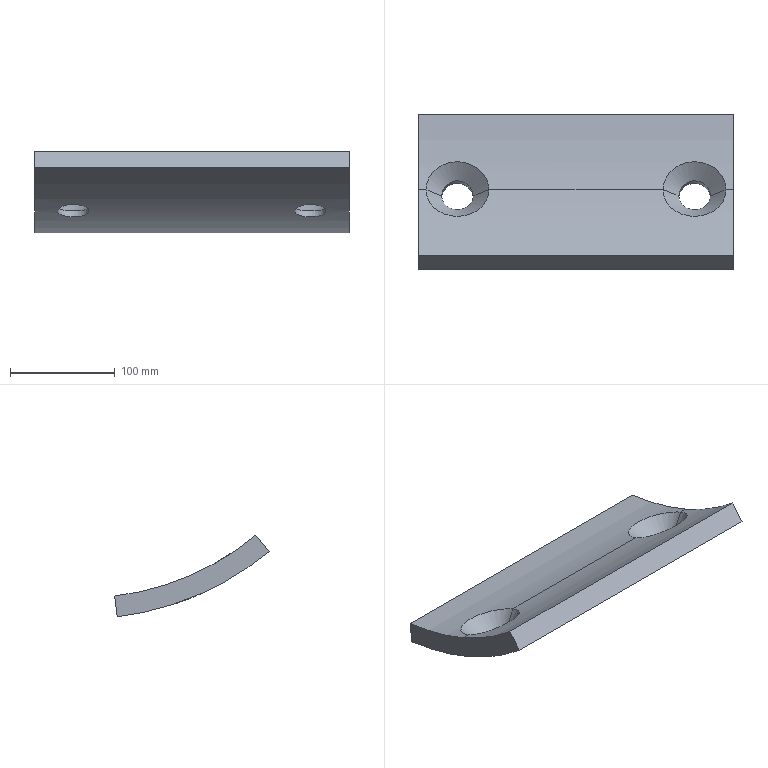Component | SolidWorks | Donja oslona ploca-10_Donja kontaktna ploca-1 | 1 solid | 16 faces | volume 872472 mm3 | cylinder 8 | spline 4 | plane 4 | commonest cylinder face diameters 30 x4 521 x2 561 x2